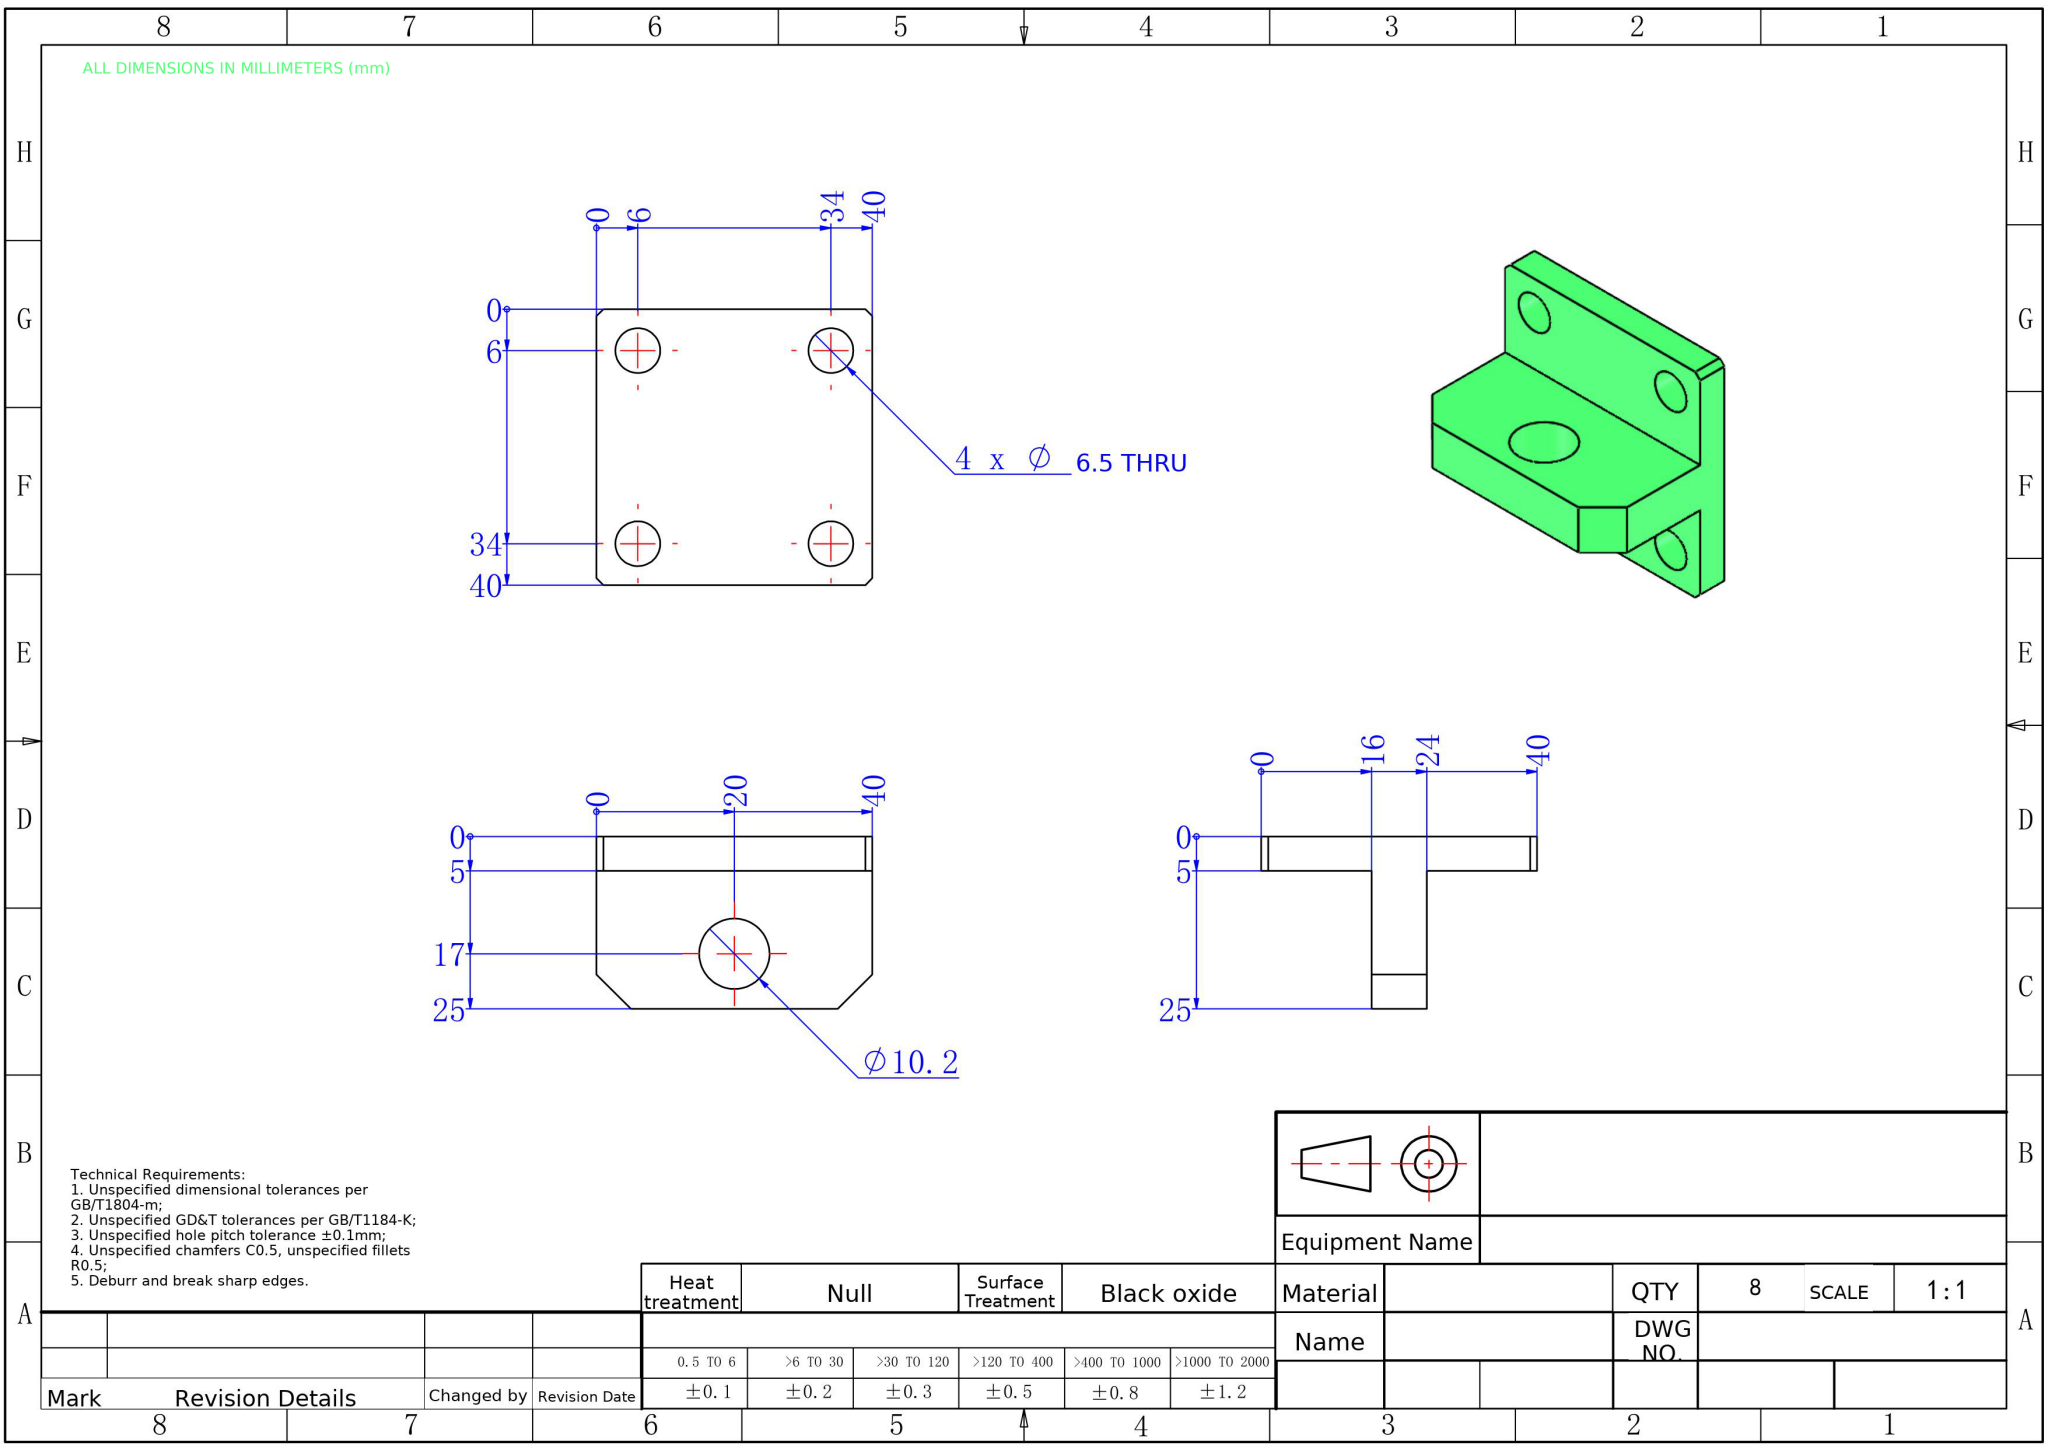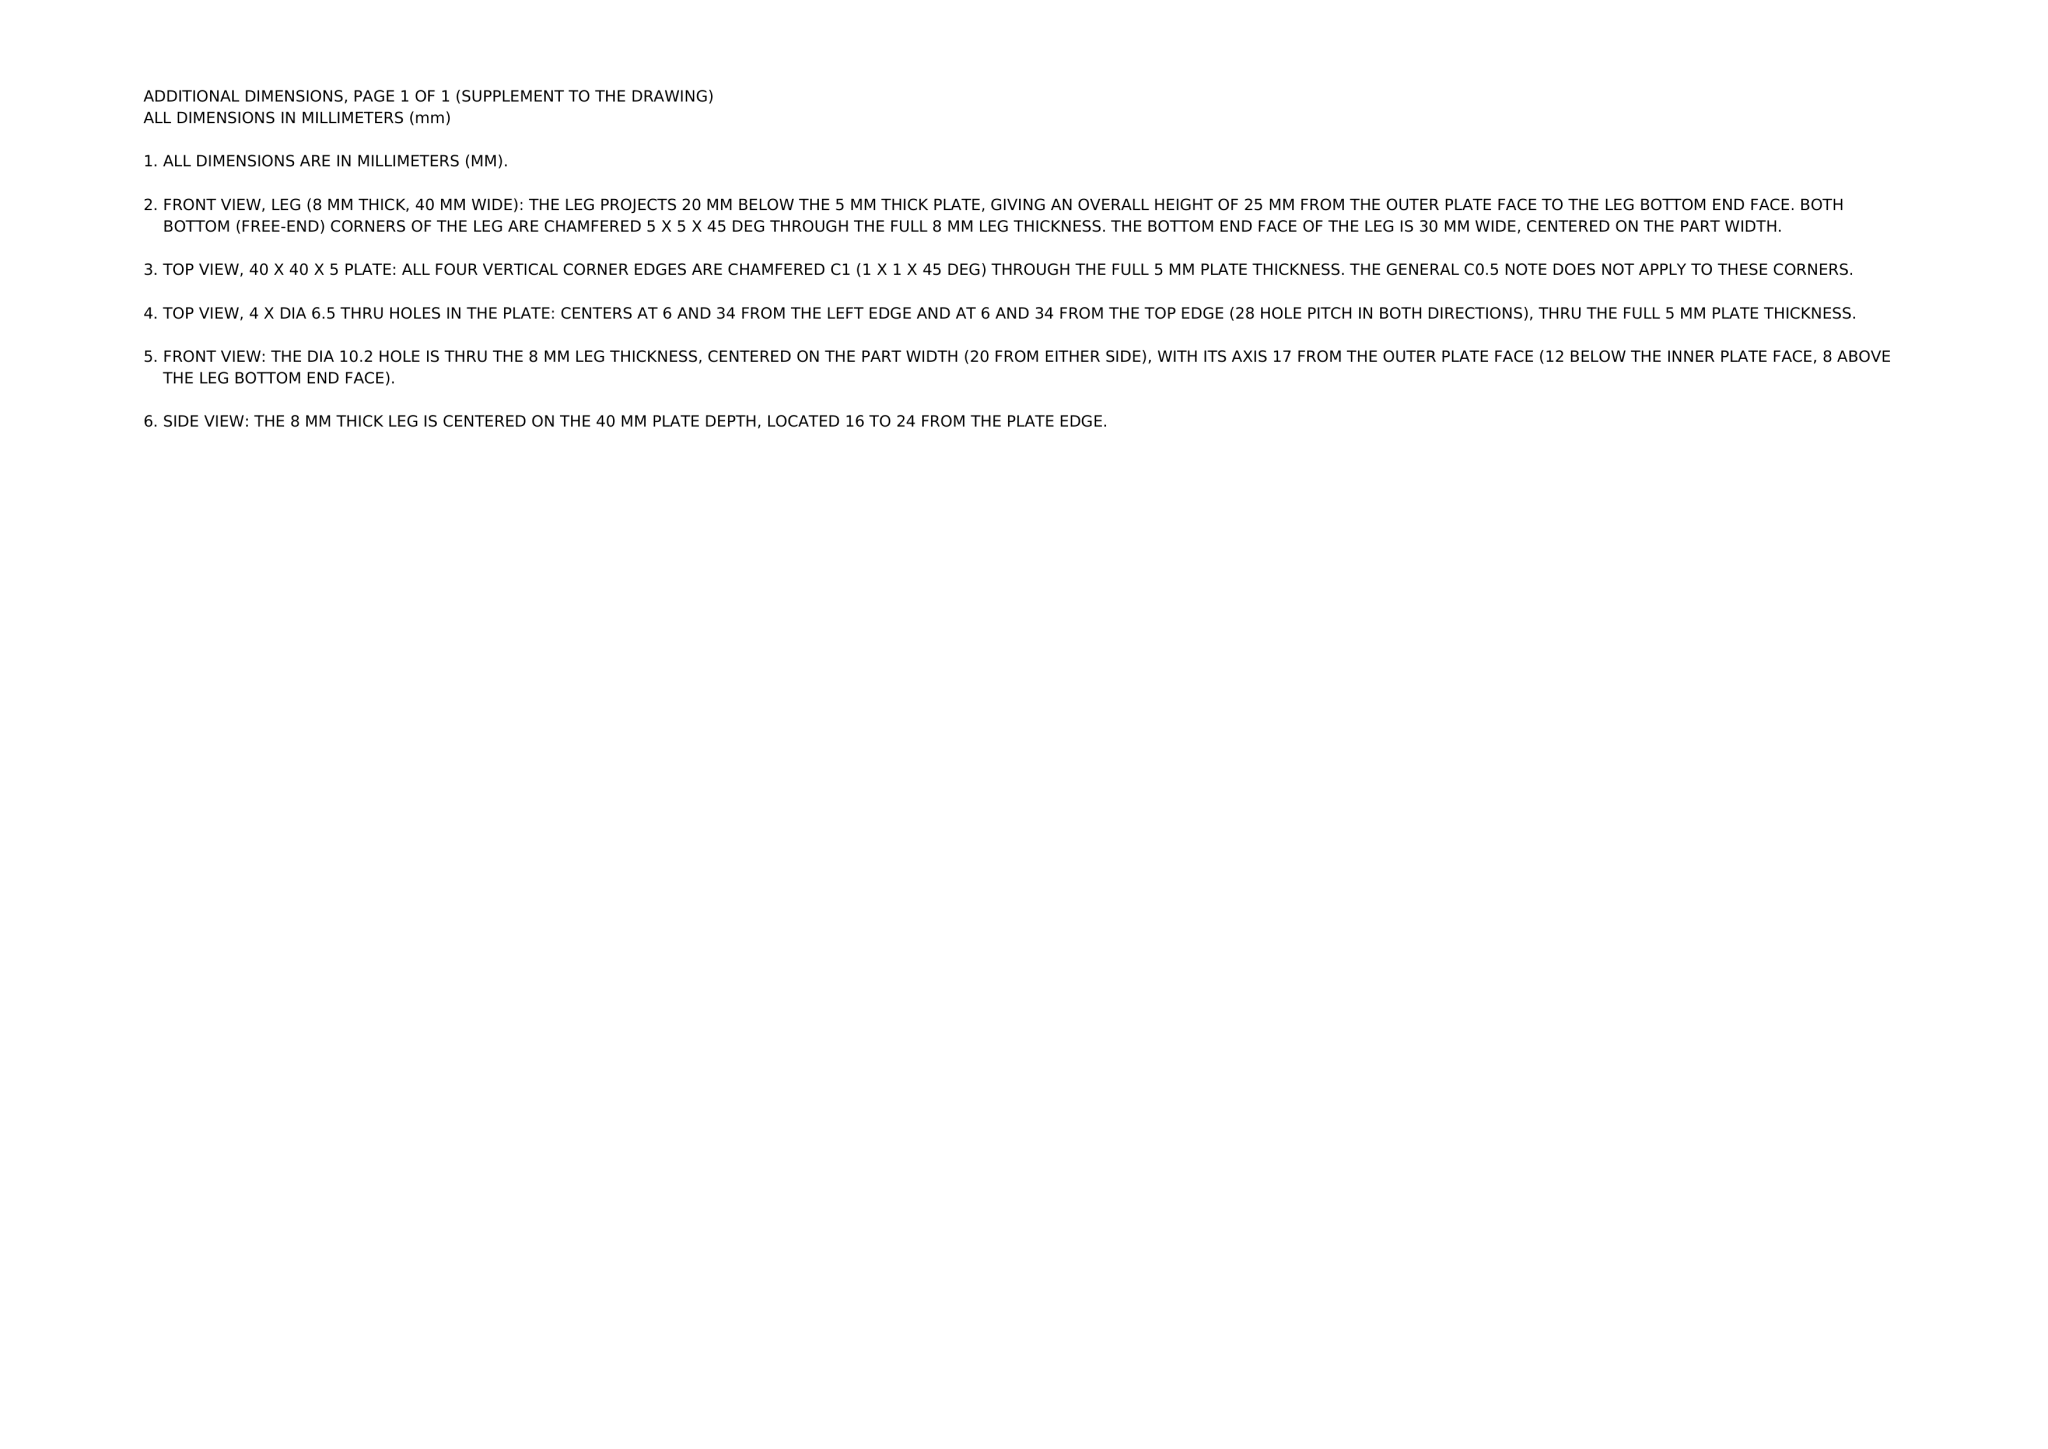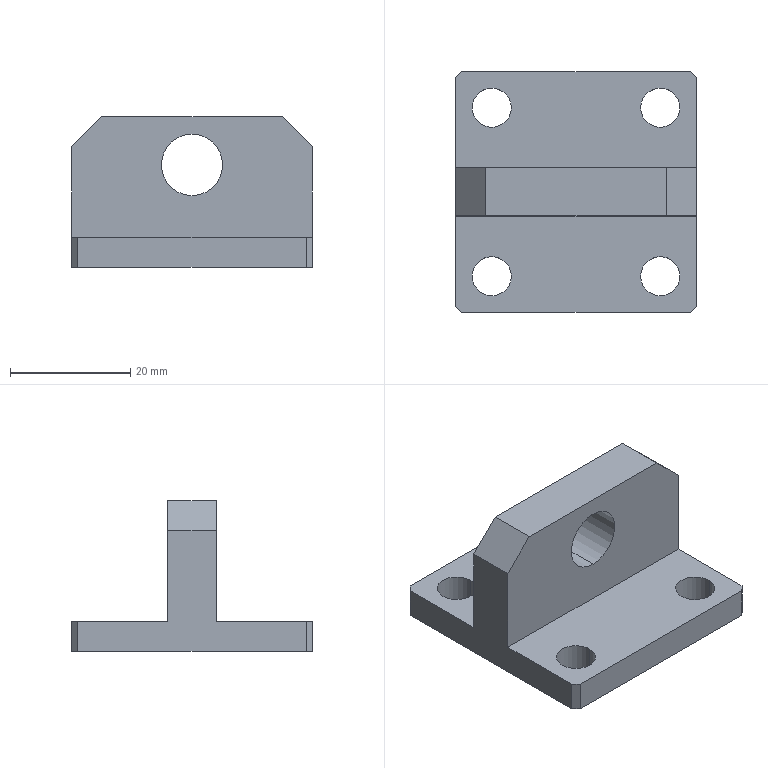Part | NX | mm | 1 solid | 26 faces | box 40 x 40 x 25 mm | volume 12873 mm3 | plane 16 | cylinder 10 | commonest cylinder face diameters 6.5 x8 10.2 x2
STEP:
#1=COLOUR_RGB('',0.7922,0.8196,0.9333);
#2=FILL_AREA_STYLE_COLOUR('',#1);
#3=FILL_AREA_STYLE('',(#2));
#4=SURFACE_STYLE_FILL_AREA(#3);
#5=SURFACE_SIDE_STYLE('',(#4));
#6=SURFACE_STYLE_USAGE(.BOTH.,#5);
#7=PRESENTATION_STYLE_ASSIGNMENT((#6));
#8=CARTESIAN_POINT('',(0.,-4.,11.9));
#9=VERTEX_POINT('',#8);
#10=CARTESIAN_POINT('',(0.,-4.,22.1));
#11=VERTEX_POINT('',#10);
#12=CARTESIAN_POINT('',(0.,-4.,17.));
#13=DIRECTION('',(0.,1.,0.));
#14=DIRECTION('',(0.,0.,1.));
#15=AXIS2_PLACEMENT_3D('',#12,#13,#14);
#16=CIRCLE('',#15,5.1);
#17=EDGE_CURVE('',#9,#11,#16,.T.);
#18=ORIENTED_EDGE('',*,*,#17,.F.);
#19=CARTESIAN_POINT('',(0.,4.,11.9));
#20=VERTEX_POINT('',#19);
#21=CARTESIAN_POINT('',(0.,-20.,11.9));
#22=DIRECTION('',(0.,1.,0.));
#23=VECTOR('',#22,1000.);
#24=LINE('',#21,#23);
#25=EDGE_CURVE('',#9,#20,#24,.T.);
#26=ORIENTED_EDGE('',*,*,#25,.T.);
#27=CARTESIAN_POINT('',(0.,4.,22.1));
#28=VERTEX_POINT('',#27);
#29=CARTESIAN_POINT('',(0.,4.,17.));
#30=DIRECTION('',(0.,1.,0.));
#31=DIRECTION('',(0.,0.,1.));
#32=AXIS2_PLACEMENT_3D('',#29,#30,#31);
#33=CIRCLE('',#32,5.1);
#34=EDGE_CURVE('',#20,#28,#33,.T.);
#35=ORIENTED_EDGE('',*,*,#34,.T.);
#36=CARTESIAN_POINT('',(0.,-20.,22.1));
#37=DIRECTION('',(0.,1.,0.));
#38=VECTOR('',#37,1000.);
#39=LINE('',#36,#38);
#40=EDGE_CURVE('',#11,#28,#39,.T.);
#41=ORIENTED_EDGE('',*,*,#40,.F.);
#42=EDGE_LOOP('',(#18,#26,#35,#41));
#43=FACE_OUTER_BOUND('',#42,.T.);
#44=CARTESIAN_POINT('',(0.,-20.,17.));
#45=DIRECTION('',(0.,1.,0.));
#46=DIRECTION('',(0.,0.,1.));
#47=AXIS2_PLACEMENT_3D('',#44,#45,#46);
#48=CYLINDRICAL_SURFACE('',#47,5.1);
#49=ADVANCED_FACE('',(#43),#48,.F.);
#50=CARTESIAN_POINT('',(10.75,-14.,0.));
#51=VERTEX_POINT('',#50);
#52=CARTESIAN_POINT('',(17.25,-14.,0.));
#53=VERTEX_POINT('',#52);
#54=CARTESIAN_POINT('',(14.,-14.,0.));
#55=DIRECTION('',(0.,0.,1.));
#56=DIRECTION('',(1.,0.,0.));
#57=AXIS2_PLACEMENT_3D('',#54,#55,#56);
#58=CIRCLE('',#57,3.25);
#59=EDGE_CURVE('',#51,#53,#58,.T.);
#60=ORIENTED_EDGE('',*,*,#59,.F.);
#61=CARTESIAN_POINT('',(10.75,-14.,5.));
#62=VERTEX_POINT('',#61);
#63=CARTESIAN_POINT('',(10.75,-14.,5.));
#64=DIRECTION('',(0.,0.,1.));
#65=VECTOR('',#64,1000.);
#66=LINE('',#63,#65);
#67=EDGE_CURVE('',#51,#62,#66,.T.);
#68=ORIENTED_EDGE('',*,*,#67,.T.);
#69=CARTESIAN_POINT('',(17.25,-14.,5.));
#70=VERTEX_POINT('',#69);
#71=CARTESIAN_POINT('',(14.,-14.,5.));
#72=DIRECTION('',(0.,0.,1.));
#73=DIRECTION('',(1.,0.,0.));
#74=AXIS2_PLACEMENT_3D('',#71,#72,#73);
#75=CIRCLE('',#74,3.25);
#76=EDGE_CURVE('',#62,#70,#75,.T.);
#77=ORIENTED_EDGE('',*,*,#76,.T.);
#78=CARTESIAN_POINT('',(17.25,-14.,5.));
#79=DIRECTION('',(0.,0.,1.));
#80=VECTOR('',#79,1000.);
#81=LINE('',#78,#80);
#82=EDGE_CURVE('',#53,#70,#81,.T.);
#83=ORIENTED_EDGE('',*,*,#82,.F.);
#84=EDGE_LOOP('',(#60,#68,#77,#83));
#85=FACE_OUTER_BOUND('',#84,.T.);
#86=CARTESIAN_POINT('',(14.,-14.,5.));
#87=DIRECTION('',(0.,0.,1.));
#88=DIRECTION('',(1.,0.,0.));
#89=AXIS2_PLACEMENT_3D('',#86,#87,#88);
#90=CYLINDRICAL_SURFACE('',#89,3.25);
#91=ADVANCED_FACE('',(#85),#90,.F.);
#92=CARTESIAN_POINT('',(-17.25,14.,0.));
#93=VERTEX_POINT('',#92);
#94=CARTESIAN_POINT('',(-10.75,14.,0.));
#95=VERTEX_POINT('',#94);
#96=CARTESIAN_POINT('',(-14.,14.,0.));
#97=DIRECTION('',(0.,0.,1.));
#98=DIRECTION('',(1.,0.,0.));
#99=AXIS2_PLACEMENT_3D('',#96,#97,#98);
#100=CIRCLE('',#99,3.25);
#101=EDGE_CURVE('',#93,#95,#100,.T.);
#102=ORIENTED_EDGE('',*,*,#101,.F.);
#103=CARTESIAN_POINT('',(-17.25,14.,5.));
#104=VERTEX_POINT('',#103);
#105=CARTESIAN_POINT('',(-17.25,14.,5.));
#106=DIRECTION('',(0.,0.,1.));
#107=VECTOR('',#106,1000.);
#108=LINE('',#105,#107);
#109=EDGE_CURVE('',#93,#104,#108,.T.);
#110=ORIENTED_EDGE('',*,*,#109,.T.);
#111=CARTESIAN_POINT('',(-10.75,14.,5.));
#112=VERTEX_POINT('',#111);
#113=CARTESIAN_POINT('',(-14.,14.,5.));
#114=DIRECTION('',(0.,0.,1.));
#115=DIRECTION('',(1.,0.,0.));
#116=AXIS2_PLACEMENT_3D('',#113,#114,#115);
#117=CIRCLE('',#116,3.25);
#118=EDGE_CURVE('',#104,#112,#117,.T.);
#119=ORIENTED_EDGE('',*,*,#118,.T.);
#120=CARTESIAN_POINT('',(-10.75,14.,5.));
#121=DIRECTION('',(0.,0.,1.));
#122=VECTOR('',#121,1000.);
#123=LINE('',#120,#122);
#124=EDGE_CURVE('',#95,#112,#123,.T.);
#125=ORIENTED_EDGE('',*,*,#124,.F.);
#126=EDGE_LOOP('',(#102,#110,#119,#125));
#127=FACE_OUTER_BOUND('',#126,.T.);
#128=CARTESIAN_POINT('',(-14.,14.,5.));
#129=DIRECTION('',(0.,0.,1.));
#130=DIRECTION('',(1.,0.,0.));
#131=AXIS2_PLACEMENT_3D('',#128,#129,#130);
#132=CYLINDRICAL_SURFACE('',#131,3.25);
#133=ADVANCED_FACE('',(#127),#132,.F.);
#134=CARTESIAN_POINT('',(-17.25,-14.,0.));
#135=VERTEX_POINT('',#134);
#136=CARTESIAN_POINT('',(-10.75,-14.,0.));
#137=VERTEX_POINT('',#136);
#138=CARTESIAN_POINT('',(-14.,-14.,0.));
#139=DIRECTION('',(0.,0.,1.));
#140=DIRECTION('',(1.,0.,0.));
#141=AXIS2_PLACEMENT_3D('',#138,#139,#140);
#142=CIRCLE('',#141,3.25);
#143=EDGE_CURVE('',#135,#137,#142,.T.);
#144=ORIENTED_EDGE('',*,*,#143,.F.);
#145=CARTESIAN_POINT('',(-17.25,-14.,5.));
#146=VERTEX_POINT('',#145);
#147=CARTESIAN_POINT('',(-17.25,-14.,5.));
#148=DIRECTION('',(0.,0.,1.));
#149=VECTOR('',#148,1000.);
#150=LINE('',#147,#149);
#151=EDGE_CURVE('',#135,#146,#150,.T.);
#152=ORIENTED_EDGE('',*,*,#151,.T.);
#153=CARTESIAN_POINT('',(-10.75,-14.,5.));
#154=VERTEX_POINT('',#153);
#155=CARTESIAN_POINT('',(-14.,-14.,5.));
#156=DIRECTION('',(0.,0.,1.));
#157=DIRECTION('',(1.,0.,0.));
#158=AXIS2_PLACEMENT_3D('',#155,#156,#157);
#159=CIRCLE('',#158,3.25);
#160=EDGE_CURVE('',#146,#154,#159,.T.);
#161=ORIENTED_EDGE('',*,*,#160,.T.);
#162=CARTESIAN_POINT('',(-10.75,-14.,5.));
#163=DIRECTION('',(0.,0.,1.));
#164=VECTOR('',#163,1000.);
#165=LINE('',#162,#164);
#166=EDGE_CURVE('',#137,#154,#165,.T.);
#167=ORIENTED_EDGE('',*,*,#166,.F.);
#168=EDGE_LOOP('',(#144,#152,#161,#167));
#169=FACE_OUTER_BOUND('',#168,.T.);
#170=CARTESIAN_POINT('',(-14.,-14.,5.));
#171=DIRECTION('',(0.,0.,1.));
#172=DIRECTION('',(1.,0.,0.));
#173=AXIS2_PLACEMENT_3D('',#170,#171,#172);
#174=CYLINDRICAL_SURFACE('',#173,3.25);
#175=ADVANCED_FACE('',(#169),#174,.F.);
#176=CARTESIAN_POINT('',(10.75,14.,0.));
#177=VERTEX_POINT('',#176);
#178=CARTESIAN_POINT('',(17.25,14.,0.));
#179=VERTEX_POINT('',#178);
#180=CARTESIAN_POINT('',(14.,14.,0.));
#181=DIRECTION('',(0.,0.,1.));
#182=DIRECTION('',(1.,0.,0.));
#183=AXIS2_PLACEMENT_3D('',#180,#181,#182);
#184=CIRCLE('',#183,3.25);
#185=EDGE_CURVE('',#177,#179,#184,.T.);
#186=ORIENTED_EDGE('',*,*,#185,.F.);
#187=CARTESIAN_POINT('',(10.75,14.,5.));
#188=VERTEX_POINT('',#187);
#189=CARTESIAN_POINT('',(10.75,14.,5.));
#190=DIRECTION('',(0.,0.,1.));
#191=VECTOR('',#190,1000.);
#192=LINE('',#189,#191);
#193=EDGE_CURVE('',#177,#188,#192,.T.);
#194=ORIENTED_EDGE('',*,*,#193,.T.);
#195=CARTESIAN_POINT('',(17.25,14.,5.));
#196=VERTEX_POINT('',#195);
#197=CARTESIAN_POINT('',(14.,14.,5.));
#198=DIRECTION('',(0.,0.,1.));
#199=DIRECTION('',(1.,0.,0.));
#200=AXIS2_PLACEMENT_3D('',#197,#198,#199);
#201=CIRCLE('',#200,3.25);
#202=EDGE_CURVE('',#188,#196,#201,.T.);
#203=ORIENTED_EDGE('',*,*,#202,.T.);
#204=CARTESIAN_POINT('',(17.25,14.,5.));
#205=DIRECTION('',(0.,0.,1.));
#206=VECTOR('',#205,1000.);
#207=LINE('',#204,#206);
#208=EDGE_CURVE('',#179,#196,#207,.T.);
#209=ORIENTED_EDGE('',*,*,#208,.F.);
#210=EDGE_LOOP('',(#186,#194,#203,#209));
#211=FACE_OUTER_BOUND('',#210,.T.);
#212=CARTESIAN_POINT('',(14.,14.,5.));
#213=DIRECTION('',(0.,0.,1.));
#214=DIRECTION('',(1.,0.,0.));
#215=AXIS2_PLACEMENT_3D('',#212,#213,#214);
#216=CYLINDRICAL_SURFACE('',#215,3.25);
#217=ADVANCED_FACE('',(#211),#216,.F.);
#218=CARTESIAN_POINT('',(-20.,-4.,5.));
#219=VERTEX_POINT('',#218);
#220=CARTESIAN_POINT('',(20.,-4.,5.));
#221=VERTEX_POINT('',#220);
#222=CARTESIAN_POINT('',(-20.,-4.,5.));
#223=DIRECTION('',(1.,0.,0.));
#224=VECTOR('',#223,1000.);
#225=LINE('',#222,#224);
#226=EDGE_CURVE('',#219,#221,#225,.T.);
#227=ORIENTED_EDGE('',*,*,#226,.F.);
#228=CARTESIAN_POINT('',(-20.,-19.,5.));
#229=VERTEX_POINT('',#228);
#230=CARTESIAN_POINT('',(-20.,20.,5.));
#231=DIRECTION('',(0.,-1.,0.));
#232=VECTOR('',#231,1000.);
#233=LINE('',#230,#232);
#234=EDGE_CURVE('',#219,#229,#233,.T.);
#235=ORIENTED_EDGE('',*,*,#234,.T.);
#236=CARTESIAN_POINT('',(-19.,-20.,5.));
#237=VERTEX_POINT('',#236);
#238=CARTESIAN_POINT('',(-19.5,-19.5,5.));
#239=DIRECTION('',(0.7071,-0.7071,0.));
#240=VECTOR('',#239,1000.);
#241=LINE('',#238,#240);
#242=EDGE_CURVE('',#229,#237,#241,.T.);
#243=ORIENTED_EDGE('',*,*,#242,.T.);
#244=CARTESIAN_POINT('',(19.,-20.,5.));
#245=VERTEX_POINT('',#244);
#246=CARTESIAN_POINT('',(-20.,-20.,5.));
#247=DIRECTION('',(1.,0.,0.));
#248=VECTOR('',#247,1000.);
#249=LINE('',#246,#248);
#250=EDGE_CURVE('',#237,#245,#249,.T.);
#251=ORIENTED_EDGE('',*,*,#250,.T.);
#252=CARTESIAN_POINT('',(20.,-19.,5.));
#253=VERTEX_POINT('',#252);
#254=CARTESIAN_POINT('',(19.5,-19.5,5.));
#255=DIRECTION('',(0.7071,0.7071,0.));
#256=VECTOR('',#255,1000.);
#257=LINE('',#254,#256);
#258=EDGE_CURVE('',#245,#253,#257,.T.);
#259=ORIENTED_EDGE('',*,*,#258,.T.);
#260=CARTESIAN_POINT('',(20.,20.,5.));
#261=DIRECTION('',(-0.,1.,0.));
#262=VECTOR('',#261,1000.);
#263=LINE('',#260,#262);
#264=EDGE_CURVE('',#253,#221,#263,.T.);
#265=ORIENTED_EDGE('',*,*,#264,.T.);
#266=EDGE_LOOP('',(#227,#235,#243,#251,#259,#265));
#267=FACE_OUTER_BOUND('',#266,.T.);
#268=CARTESIAN_POINT('',(-14.,-14.,5.));
#269=DIRECTION('',(0.,0.,1.));
#270=DIRECTION('',(1.,0.,0.));
#271=AXIS2_PLACEMENT_3D('',#268,#269,#270);
#272=CIRCLE('',#271,3.25);
#273=EDGE_CURVE('',#154,#146,#272,.T.);
#274=ORIENTED_EDGE('',*,*,#273,.F.);
#275=ORIENTED_EDGE('',*,*,#160,.F.);
#276=EDGE_LOOP('',(#274,#275));
#277=FACE_BOUND('',#276,.T.);
#278=CARTESIAN_POINT('',(14.,-14.,5.));
#279=DIRECTION('',(0.,0.,1.));
#280=DIRECTION('',(1.,0.,0.));
#281=AXIS2_PLACEMENT_3D('',#278,#279,#280);
#282=CIRCLE('',#281,3.25);
#283=EDGE_CURVE('',#70,#62,#282,.T.);
#284=ORIENTED_EDGE('',*,*,#283,.F.);
#285=ORIENTED_EDGE('',*,*,#76,.F.);
#286=EDGE_LOOP('',(#284,#285));
#287=FACE_BOUND('',#286,.T.);
#288=CARTESIAN_POINT('',(0.,0.,5.));
#289=DIRECTION('',(0.,0.,1.));
#290=DIRECTION('',(1.,0.,0.));
#291=AXIS2_PLACEMENT_3D('',#288,#289,#290);
#292=PLANE('',#291);
#293=ADVANCED_FACE('',(#267,#277,#287),#292,.T.);
#294=CARTESIAN_POINT('',(20.,4.,20.));
#295=VERTEX_POINT('',#294);
#296=CARTESIAN_POINT('',(20.,4.,5.));
#297=VERTEX_POINT('',#296);
#298=CARTESIAN_POINT('',(20.,4.,25.));
#299=DIRECTION('',(0.,0.,-1.));
#300=VECTOR('',#299,1000.);
#301=LINE('',#298,#300);
#302=EDGE_CURVE('',#295,#297,#301,.T.);
#303=ORIENTED_EDGE('',*,*,#302,.F.);
#304=CARTESIAN_POINT('',(20.,-4.,20.));
#305=VERTEX_POINT('',#304);
#306=CARTESIAN_POINT('',(20.,-4.,20.));
#307=DIRECTION('',(0.,-1.,0.));
#308=VECTOR('',#307,1000.);
#309=LINE('',#306,#308);
#310=EDGE_CURVE('',#295,#305,#309,.T.);
#311=ORIENTED_EDGE('',*,*,#310,.T.);
#312=CARTESIAN_POINT('',(20.,-4.,25.));
#313=DIRECTION('',(0.,0.,-1.));
#314=VECTOR('',#313,1000.);
#315=LINE('',#312,#314);
#316=EDGE_CURVE('',#305,#221,#315,.T.);
#317=ORIENTED_EDGE('',*,*,#316,.T.);
#318=ORIENTED_EDGE('',*,*,#264,.F.);
#319=CARTESIAN_POINT('',(20.,-19.,0.));
#320=VERTEX_POINT('',#319);
#321=CARTESIAN_POINT('',(20.,-19.,5.));
#322=DIRECTION('',(0.,0.,-1.));
#323=VECTOR('',#322,1000.);
#324=LINE('',#321,#323);
#325=EDGE_CURVE('',#253,#320,#324,.T.);
#326=ORIENTED_EDGE('',*,*,#325,.T.);
#327=CARTESIAN_POINT('',(20.,19.,0.));
#328=VERTEX_POINT('',#327);
#329=CARTESIAN_POINT('',(20.,20.,0.));
#330=DIRECTION('',(-0.,1.,0.));
#331=VECTOR('',#330,1000.);
#332=LINE('',#329,#331);
#333=EDGE_CURVE('',#320,#328,#332,.T.);
#334=ORIENTED_EDGE('',*,*,#333,.T.);
#335=CARTESIAN_POINT('',(20.,19.,5.));
#336=VERTEX_POINT('',#335);
#337=CARTESIAN_POINT('',(20.,19.,5.));
#338=DIRECTION('',(0.,0.,1.));
#339=VECTOR('',#338,1000.);
#340=LINE('',#337,#339);
#341=EDGE_CURVE('',#328,#336,#340,.T.);
#342=ORIENTED_EDGE('',*,*,#341,.T.);
#343=CARTESIAN_POINT('',(20.,20.,5.));
#344=DIRECTION('',(-0.,1.,0.));
#345=VECTOR('',#344,1000.);
#346=LINE('',#343,#345);
#347=EDGE_CURVE('',#297,#336,#346,.T.);
#348=ORIENTED_EDGE('',*,*,#347,.F.);
#349=EDGE_LOOP('',(#303,#311,#317,#318,#326,#334,#342,#348));
#350=FACE_OUTER_BOUND('',#349,.T.);
#351=CARTESIAN_POINT('',(20.,20.,5.));
#352=DIRECTION('',(-1.,-0.,0.));
#353=DIRECTION('',(0.,-1.,0.));
#354=AXIS2_PLACEMENT_3D('',#351,#352,#353);
#355=PLANE('',#354);
#356=ADVANCED_FACE('',(#350),#355,.F.);
#357=CARTESIAN_POINT('',(19.,20.,0.));
#358=VERTEX_POINT('',#357);
#359=CARTESIAN_POINT('',(-19.,20.,0.));
#360=VERTEX_POINT('',#359);
#361=CARTESIAN_POINT('',(-20.,20.,0.));
#362=DIRECTION('',(-1.,0.,0.));
#363=VECTOR('',#362,1000.);
#364=LINE('',#361,#363);
#365=EDGE_CURVE('',#358,#360,#364,.T.);
#366=ORIENTED_EDGE('',*,*,#365,.T.);
#367=CARTESIAN_POINT('',(-19.,20.,5.));
#368=VERTEX_POINT('',#367);
#369=CARTESIAN_POINT('',(-19.,20.,5.));
#370=DIRECTION('',(0.,0.,1.));
#371=VECTOR('',#370,1000.);
#372=LINE('',#369,#371);
#373=EDGE_CURVE('',#360,#368,#372,.T.);
#374=ORIENTED_EDGE('',*,*,#373,.T.);
#375=CARTESIAN_POINT('',(19.,20.,5.));
#376=VERTEX_POINT('',#375);
#377=CARTESIAN_POINT('',(-20.,20.,5.));
#378=DIRECTION('',(-1.,0.,0.));
#379=VECTOR('',#378,1000.);
#380=LINE('',#377,#379);
#381=EDGE_CURVE('',#376,#368,#380,.T.);
#382=ORIENTED_EDGE('',*,*,#381,.F.);
#383=CARTESIAN_POINT('',(19.,20.,5.));
#384=DIRECTION('',(0.,0.,-1.));
#385=VECTOR('',#384,1000.);
#386=LINE('',#383,#385);
#387=EDGE_CURVE('',#376,#358,#386,.T.);
#388=ORIENTED_EDGE('',*,*,#387,.T.);
#389=EDGE_LOOP('',(#366,#374,#382,#388));
#390=FACE_OUTER_BOUND('',#389,.T.);
#391=CARTESIAN_POINT('',(-20.,20.,5.));
#392=DIRECTION('',(0.,-1.,0.));
#393=DIRECTION('',(0.,0.,-1.));
#394=AXIS2_PLACEMENT_3D('',#391,#392,#393);
#395=PLANE('',#394);
#396=ADVANCED_FACE('',(#390),#395,.F.);
#397=CARTESIAN_POINT('',(-20.,-4.,20.));
#398=VERTEX_POINT('',#397);
#399=CARTESIAN_POINT('',(-20.,-4.,25.));
#400=DIRECTION('',(0.,0.,-1.));
#401=VECTOR('',#400,1000.);
#402=LINE('',#399,#401);
#403=EDGE_CURVE('',#398,#219,#402,.T.);
#404=ORIENTED_EDGE('',*,*,#403,.F.);
#405=CARTESIAN_POINT('',(-20.,4.,20.));
#406=VERTEX_POINT('',#405);
#407=CARTESIAN_POINT('',(-20.,4.,20.));
#408=DIRECTION('',(-0.,1.,0.));
#409=VECTOR('',#408,1000.);
#410=LINE('',#407,#409);
#411=EDGE_CURVE('',#398,#406,#410,.T.);
#412=ORIENTED_EDGE('',*,*,#411,.T.);
#413=CARTESIAN_POINT('',(-20.,4.,5.));
#414=VERTEX_POINT('',#413);
#415=CARTESIAN_POINT('',(-20.,4.,25.));
#416=DIRECTION('',(0.,0.,-1.));
#417=VECTOR('',#416,1000.);
#418=LINE('',#415,#417);
#419=EDGE_CURVE('',#406,#414,#418,.T.);
#420=ORIENTED_EDGE('',*,*,#419,.T.);
#421=CARTESIAN_POINT('',(-20.,19.,5.));
#422=VERTEX_POINT('',#421);
#423=CARTESIAN_POINT('',(-20.,20.,5.));
#424=DIRECTION('',(0.,-1.,0.));
#425=VECTOR('',#424,1000.);
#426=LINE('',#423,#425);
#427=EDGE_CURVE('',#422,#414,#426,.T.);
#428=ORIENTED_EDGE('',*,*,#427,.F.);
#429=CARTESIAN_POINT('',(-20.,19.,0.));
#430=VERTEX_POINT('',#429);
#431=CARTESIAN_POINT('',(-20.,19.,5.));
#432=DIRECTION('',(0.,0.,-1.));
#433=VECTOR('',#432,1000.);
#434=LINE('',#431,#433);
#435=EDGE_CURVE('',#422,#430,#434,.T.);
#436=ORIENTED_EDGE('',*,*,#435,.T.);
#437=CARTESIAN_POINT('',(-20.,-19.,0.));
#438=VERTEX_POINT('',#437);
#439=CARTESIAN_POINT('',(-20.,20.,0.));
#440=DIRECTION('',(0.,-1.,0.));
#441=VECTOR('',#440,1000.);
#442=LINE('',#439,#441);
#443=EDGE_CURVE('',#430,#438,#442,.T.);
#444=ORIENTED_EDGE('',*,*,#443,.T.);
#445=CARTESIAN_POINT('',(-20.,-19.,5.));
#446=DIRECTION('',(0.,0.,1.));
#447=VECTOR('',#446,1000.);
#448=LINE('',#445,#447);
#449=EDGE_CURVE('',#438,#229,#448,.T.);
#450=ORIENTED_EDGE('',*,*,#449,.T.);
#451=ORIENTED_EDGE('',*,*,#234,.F.);
#452=EDGE_LOOP('',(#404,#412,#420,#428,#436,#444,#450,#451));
#453=FACE_OUTER_BOUND('',#452,.T.);
#454=CARTESIAN_POINT('',(-20.,20.,5.));
#455=DIRECTION('',(1.,0.,0.));
#456=DIRECTION('',(-0.,1.,0.));
#457=AXIS2_PLACEMENT_3D('',#454,#455,#456);
#458=PLANE('',#457);
#459=ADVANCED_FACE('',(#453),#458,.F.);
#460=ORIENTED_EDGE('',*,*,#250,.F.);
#461=CARTESIAN_POINT('',(-19.,-20.,0.));
#462=VERTEX_POINT('',#461);
#463=CARTESIAN_POINT('',(-19.,-20.,5.));
#464=DIRECTION('',(0.,0.,-1.));
#465=VECTOR('',#464,1000.);
#466=LINE('',#463,#465);
#467=EDGE_CURVE('',#237,#462,#466,.T.);
#468=ORIENTED_EDGE('',*,*,#467,.T.);
#469=CARTESIAN_POINT('',(19.,-20.,0.));
#470=VERTEX_POINT('',#469);
#471=CARTESIAN_POINT('',(-20.,-20.,0.));
#472=DIRECTION('',(1.,0.,0.));
#473=VECTOR('',#472,1000.);
#474=LINE('',#471,#473);
#475=EDGE_CURVE('',#462,#470,#474,.T.);
#476=ORIENTED_EDGE('',*,*,#475,.T.);
#477=CARTESIAN_POINT('',(19.,-20.,5.));
#478=DIRECTION('',(0.,0.,1.));
#479=VECTOR('',#478,1000.);
#480=LINE('',#477,#479);
#481=EDGE_CURVE('',#470,#245,#480,.T.);
#482=ORIENTED_EDGE('',*,*,#481,.T.);
#483=EDGE_LOOP('',(#460,#468,#476,#482));
#484=FACE_OUTER_BOUND('',#483,.T.);
#485=CARTESIAN_POINT('',(-20.,-20.,5.));
#486=DIRECTION('',(0.,1.,0.));
#487=DIRECTION('',(0.,0.,1.));
#488=AXIS2_PLACEMENT_3D('',#485,#486,#487);
#489=PLANE('',#488);
#490=ADVANCED_FACE('',(#484),#489,.F.);
#491=CARTESIAN_POINT('',(-20.,4.,5.));
#492=DIRECTION('',(-1.,0.,0.));
#493=VECTOR('',#492,1000.);
#494=LINE('',#491,#493);
#495=EDGE_CURVE('',#297,#414,#494,.T.);
#496=ORIENTED_EDGE('',*,*,#495,.F.);
#497=ORIENTED_EDGE('',*,*,#347,.T.);
#498=CARTESIAN_POINT('',(19.5,19.5,5.));
#499=DIRECTION('',(-0.7071,0.7071,0.));
#500=VECTOR('',#499,1000.);
#501=LINE('',#498,#500);
#502=EDGE_CURVE('',#336,#376,#501,.T.);
#503=ORIENTED_EDGE('',*,*,#502,.T.);
#504=ORIENTED_EDGE('',*,*,#381,.T.);
#505=CARTESIAN_POINT('',(-19.5,19.5,5.));
#506=DIRECTION('',(-0.7071,-0.7071,0.));
#507=VECTOR('',#506,1000.);
#508=LINE('',#505,#507);
#509=EDGE_CURVE('',#368,#422,#508,.T.);
#510=ORIENTED_EDGE('',*,*,#509,.T.);
#511=ORIENTED_EDGE('',*,*,#427,.T.);
#512=EDGE_LOOP('',(#496,#497,#503,#504,#510,#511));
#513=FACE_OUTER_BOUND('',#512,.T.);
#514=CARTESIAN_POINT('',(-14.,14.,5.));
#515=DIRECTION('',(0.,0.,1.));
#516=DIRECTION('',(1.,0.,0.));
#517=AXIS2_PLACEMENT_3D('',#514,#515,#516);
#518=CIRCLE('',#517,3.25);
#519=EDGE_CURVE('',#112,#104,#518,.T.);
#520=ORIENTED_EDGE('',*,*,#519,.F.);
#521=ORIENTED_EDGE('',*,*,#118,.F.);
#522=EDGE_LOOP('',(#520,#521));
#523=FACE_BOUND('',#522,.T.);
#524=CARTESIAN_POINT('',(14.,14.,5.));
#525=DIRECTION('',(0.,0.,1.));
#526=DIRECTION('',(1.,0.,0.));
#527=AXIS2_PLACEMENT_3D('',#524,#525,#526);
#528=CIRCLE('',#527,3.25);
#529=EDGE_CURVE('',#196,#188,#528,.T.);
#530=ORIENTED_EDGE('',*,*,#529,.F.);
#531=ORIENTED_EDGE('',*,*,#202,.F.);
#532=EDGE_LOOP('',(#530,#531));
#533=FACE_BOUND('',#532,.T.);
#534=CARTESIAN_POINT('',(0.,0.,5.));
#535=DIRECTION('',(0.,0.,1.));
#536=DIRECTION('',(1.,0.,0.));
#537=AXIS2_PLACEMENT_3D('',#534,#535,#536);
#538=PLANE('',#537);
#539=ADVANCED_FACE('',(#513,#523,#533),#538,.T.);
#540=CARTESIAN_POINT('',(14.,-14.,0.));
#541=DIRECTION('',(0.,0.,1.));
#542=DIRECTION('',(1.,0.,0.));
#543=AXIS2_PLACEMENT_3D('',#540,#541,#542);
#544=CIRCLE('',#543,3.25);
#545=EDGE_CURVE('',#53,#51,#544,.T.);
#546=ORIENTED_EDGE('',*,*,#545,.T.);
#547=ORIENTED_EDGE('',*,*,#59,.T.);
#548=EDGE_LOOP('',(#546,#547));
#549=FACE_BOUND('',#548,.T.);
#550=CARTESIAN_POINT('',(-14.,14.,0.));
#551=DIRECTION('',(0.,0.,1.));
#552=DIRECTION('',(1.,0.,0.));
#553=AXIS2_PLACEMENT_3D('',#550,#551,#552);
#554=CIRCLE('',#553,3.25);
#555=EDGE_CURVE('',#95,#93,#554,.T.);
#556=ORIENTED_EDGE('',*,*,#555,.T.);
#557=ORIENTED_EDGE('',*,*,#101,.T.);
#558=EDGE_LOOP('',(#556,#557));
#559=FACE_BOUND('',#558,.T.);
#560=CARTESIAN_POINT('',(-14.,-14.,0.));
#561=DIRECTION('',(0.,0.,1.));
#562=DIRECTION('',(1.,0.,0.));
#563=AXIS2_PLACEMENT_3D('',#560,#561,#562);
#564=CIRCLE('',#563,3.25);
#565=EDGE_CURVE('',#137,#135,#564,.T.);
#566=ORIENTED_EDGE('',*,*,#565,.T.);
#567=ORIENTED_EDGE('',*,*,#143,.T.);
#568=EDGE_LOOP('',(#566,#567));
#569=FACE_BOUND('',#568,.T.);
#570=CARTESIAN_POINT('',(14.,14.,0.));
#571=DIRECTION('',(0.,0.,1.));
#572=DIRECTION('',(1.,0.,0.));
#573=AXIS2_PLACEMENT_3D('',#570,#571,#572);
#574=CIRCLE('',#573,3.25);
#575=EDGE_CURVE('',#179,#177,#574,.T.);
#576=ORIENTED_EDGE('',*,*,#575,.T.);
#577=ORIENTED_EDGE('',*,*,#185,.T.);
#578=EDGE_LOOP('',(#576,#577));
#579=FACE_BOUND('',#578,.T.);
#580=ORIENTED_EDGE('',*,*,#475,.F.);
#581=CARTESIAN_POINT('',(-19.,-20.,0.));
#582=DIRECTION('',(-0.7071,0.7071,0.));
#583=VECTOR('',#582,1000.);
#584=LINE('',#581,#583);
#585=EDGE_CURVE('',#462,#438,#584,.T.);
#586=ORIENTED_EDGE('',*,*,#585,.T.);
#587=ORIENTED_EDGE('',*,*,#443,.F.);
#588=CARTESIAN_POINT('',(-20.,19.,0.));
#589=DIRECTION('',(0.7071,0.7071,0.));
#590=VECTOR('',#589,1000.);
#591=LINE('',#588,#590);
#592=EDGE_CURVE('',#430,#360,#591,.T.);
#593=ORIENTED_EDGE('',*,*,#592,.T.);
#594=ORIENTED_EDGE('',*,*,#365,.F.);
#595=CARTESIAN_POINT('',(19.,20.,0.));
#596=DIRECTION('',(0.7071,-0.7071,0.));
#597=VECTOR('',#596,1000.);
#598=LINE('',#595,#597);
#599=EDGE_CURVE('',#358,#328,#598,.T.);
#600=ORIENTED_EDGE('',*,*,#599,.T.);
#601=ORIENTED_EDGE('',*,*,#333,.F.);
#602=CARTESIAN_POINT('',(20.,-19.,0.));
#603=DIRECTION('',(-0.7071,-0.7071,0.));
#604=VECTOR('',#603,1000.);
#605=LINE('',#602,#604);
#606=EDGE_CURVE('',#320,#470,#605,.T.);
#607=ORIENTED_EDGE('',*,*,#606,.T.);
#608=EDGE_LOOP('',(#580,#586,#587,#593,#594,#600,#601,#607));
#609=FACE_OUTER_BOUND('',#608,.T.);
#610=CARTESIAN_POINT('',(0.,0.,0.));
#611=DIRECTION('',(0.,0.,1.));
#612=DIRECTION('',(1.,0.,0.));
#613=AXIS2_PLACEMENT_3D('',#610,#611,#612);
#614=PLANE('',#613);
#615=ADVANCED_FACE('',(#549,#559,#569,#579,#609),#614,.F.);
#616=ORIENTED_EDGE('',*,*,#193,.F.);
#617=ORIENTED_EDGE('',*,*,#575,.F.);
#618=ORIENTED_EDGE('',*,*,#208,.T.);
#619=ORIENTED_EDGE('',*,*,#529,.T.);
#620=EDGE_LOOP('',(#616,#617,#618,#619));
#621=FACE_OUTER_BOUND('',#620,.T.);
#622=CARTESIAN_POINT('',(14.,14.,5.));
#623=DIRECTION('',(0.,0.,1.));
#624=DIRECTION('',(1.,0.,0.));
#625=AXIS2_PLACEMENT_3D('',#622,#623,#624);
#626=CYLINDRICAL_SURFACE('',#625,3.25);
#627=ADVANCED_FACE('',(#621),#626,.F.);
#628=ORIENTED_EDGE('',*,*,#151,.F.);
#629=ORIENTED_EDGE('',*,*,#565,.F.);
#630=ORIENTED_EDGE('',*,*,#166,.T.);
#631=ORIENTED_EDGE('',*,*,#273,.T.);
#632=EDGE_LOOP('',(#628,#629,#630,#631));
#633=FACE_OUTER_BOUND('',#632,.T.);
#634=CARTESIAN_POINT('',(-14.,-14.,5.));
#635=DIRECTION('',(0.,0.,1.));
#636=DIRECTION('',(1.,0.,0.));
#637=AXIS2_PLACEMENT_3D('',#634,#635,#636);
#638=CYLINDRICAL_SURFACE('',#637,3.25);
#639=ADVANCED_FACE('',(#633),#638,.F.);
#640=ORIENTED_EDGE('',*,*,#109,.F.);
#641=ORIENTED_EDGE('',*,*,#555,.F.);
#642=ORIENTED_EDGE('',*,*,#124,.T.);
#643=ORIENTED_EDGE('',*,*,#519,.T.);
#644=EDGE_LOOP('',(#640,#641,#642,#643));
#645=FACE_OUTER_BOUND('',#644,.T.);
#646=CARTESIAN_POINT('',(-14.,14.,5.));
#647=DIRECTION('',(0.,0.,1.));
#648=DIRECTION('',(1.,0.,0.));
#649=AXIS2_PLACEMENT_3D('',#646,#647,#648);
#650=CYLINDRICAL_SURFACE('',#649,3.25);
#651=ADVANCED_FACE('',(#645),#650,.F.);
#652=ORIENTED_EDGE('',*,*,#67,.F.);
#653=ORIENTED_EDGE('',*,*,#545,.F.);
#654=ORIENTED_EDGE('',*,*,#82,.T.);
#655=ORIENTED_EDGE('',*,*,#283,.T.);
#656=EDGE_LOOP('',(#652,#653,#654,#655));
#657=FACE_OUTER_BOUND('',#656,.T.);
#658=CARTESIAN_POINT('',(14.,-14.,5.));
#659=DIRECTION('',(0.,0.,1.));
#660=DIRECTION('',(1.,0.,0.));
#661=AXIS2_PLACEMENT_3D('',#658,#659,#660);
#662=CYLINDRICAL_SURFACE('',#661,3.25);
#663=ADVANCED_FACE('',(#657),#662,.F.);
#664=ORIENTED_EDGE('',*,*,#242,.F.);
#665=ORIENTED_EDGE('',*,*,#449,.F.);
#666=ORIENTED_EDGE('',*,*,#585,.F.);
#667=ORIENTED_EDGE('',*,*,#467,.F.);
#668=EDGE_LOOP('',(#664,#665,#666,#667));
#669=FACE_OUTER_BOUND('',#668,.T.);
#670=CARTESIAN_POINT('',(-19.,-20.,5.));
#671=DIRECTION('',(0.7071,0.7071,0.));
#672=DIRECTION('',(0.,0.,-1.));
#673=AXIS2_PLACEMENT_3D('',#670,#671,#672);
#674=PLANE('',#673);
#675=ADVANCED_FACE('',(#669),#674,.F.);
#676=ORIENTED_EDGE('',*,*,#509,.F.);
#677=ORIENTED_EDGE('',*,*,#373,.F.);
#678=ORIENTED_EDGE('',*,*,#592,.F.);
#679=ORIENTED_EDGE('',*,*,#435,.F.);
#680=EDGE_LOOP('',(#676,#677,#678,#679));
#681=FACE_OUTER_BOUND('',#680,.T.);
#682=CARTESIAN_POINT('',(-20.,19.,5.));
#683=DIRECTION('',(0.7071,-0.7071,0.));
#684=DIRECTION('',(0.,0.,-1.));
#685=AXIS2_PLACEMENT_3D('',#682,#683,#684);
#686=PLANE('',#685);
#687=ADVANCED_FACE('',(#681),#686,.F.);
#688=ORIENTED_EDGE('',*,*,#258,.F.);
#689=ORIENTED_EDGE('',*,*,#481,.F.);
#690=ORIENTED_EDGE('',*,*,#606,.F.);
#691=ORIENTED_EDGE('',*,*,#325,.F.);
#692=EDGE_LOOP('',(#688,#689,#690,#691));
#693=FACE_OUTER_BOUND('',#692,.T.);
#694=CARTESIAN_POINT('',(20.,-19.,5.));
#695=DIRECTION('',(-0.7071,0.7071,0.));
#696=DIRECTION('',(0.,0.,-1.));
#697=AXIS2_PLACEMENT_3D('',#694,#695,#696);
#698=PLANE('',#697);
#699=ADVANCED_FACE('',(#693),#698,.F.);
#700=ORIENTED_EDGE('',*,*,#502,.F.);
#701=ORIENTED_EDGE('',*,*,#341,.F.);
#702=ORIENTED_EDGE('',*,*,#599,.F.);
#703=ORIENTED_EDGE('',*,*,#387,.F.);
#704=EDGE_LOOP('',(#700,#701,#702,#703));
#705=FACE_OUTER_BOUND('',#704,.T.);
#706=CARTESIAN_POINT('',(19.,20.,5.));
#707=DIRECTION('',(-0.7071,-0.7071,0.));
#708=DIRECTION('',(0.,0.,-1.));
#709=AXIS2_PLACEMENT_3D('',#706,#707,#708);
#710=PLANE('',#709);
#711=ADVANCED_FACE('',(#705),#710,.F.);
#712=CARTESIAN_POINT('',(0.,4.,17.));
#713=DIRECTION('',(0.,1.,0.));
#714=DIRECTION('',(0.,0.,1.));
#715=AXIS2_PLACEMENT_3D('',#712,#713,#714);
#716=CIRCLE('',#715,5.1);
#717=EDGE_CURVE('',#28,#20,#716,.T.);
#718=ORIENTED_EDGE('',*,*,#717,.F.);
#719=ORIENTED_EDGE('',*,*,#34,.F.);
#720=EDGE_LOOP('',(#718,#719));
#721=FACE_BOUND('',#720,.T.);
#722=ORIENTED_EDGE('',*,*,#419,.F.);
#723=CARTESIAN_POINT('',(-15.,4.,25.));
#724=VERTEX_POINT('',#723);
#725=CARTESIAN_POINT('',(-15.,4.,25.));
#726=DIRECTION('',(0.7071,0.,0.7071));
#727=VECTOR('',#726,1000.);
#728=LINE('',#725,#727);
#729=EDGE_CURVE('',#406,#724,#728,.T.);
#730=ORIENTED_EDGE('',*,*,#729,.T.);
#731=CARTESIAN_POINT('',(15.,4.,25.));
#732=VERTEX_POINT('',#731);
#733=CARTESIAN_POINT('',(-20.,4.,25.));
#734=DIRECTION('',(-1.,0.,0.));
#735=VECTOR('',#734,1000.);
#736=LINE('',#733,#735);
#737=EDGE_CURVE('',#732,#724,#736,.T.);
#738=ORIENTED_EDGE('',*,*,#737,.F.);
#739=CARTESIAN_POINT('',(15.,4.,25.));
#740=DIRECTION('',(0.7071,0.,-0.7071));
#741=VECTOR('',#740,1000.);
#742=LINE('',#739,#741);
#743=EDGE_CURVE('',#732,#295,#742,.T.);
#744=ORIENTED_EDGE('',*,*,#743,.T.);
#745=ORIENTED_EDGE('',*,*,#302,.T.);
#746=ORIENTED_EDGE('',*,*,#495,.T.);
#747=EDGE_LOOP('',(#722,#730,#738,#744,#745,#746));
#748=FACE_OUTER_BOUND('',#747,.T.);
#749=CARTESIAN_POINT('',(-20.,4.,25.));
#750=DIRECTION('',(0.,-1.,0.));
#751=DIRECTION('',(0.,0.,-1.));
#752=AXIS2_PLACEMENT_3D('',#749,#750,#751);
#753=PLANE('',#752);
#754=ADVANCED_FACE('',(#721,#748),#753,.F.);
#755=CARTESIAN_POINT('',(0.,-4.,17.));
#756=DIRECTION('',(0.,1.,0.));
#757=DIRECTION('',(0.,0.,1.));
#758=AXIS2_PLACEMENT_3D('',#755,#756,#757);
#759=CIRCLE('',#758,5.1);
#760=EDGE_CURVE('',#11,#9,#759,.T.);
#761=ORIENTED_EDGE('',*,*,#760,.T.);
#762=ORIENTED_EDGE('',*,*,#17,.T.);
#763=EDGE_LOOP('',(#761,#762));
#764=FACE_BOUND('',#763,.T.);
#765=CARTESIAN_POINT('',(-15.,-4.,25.));
#766=VERTEX_POINT('',#765);
#767=CARTESIAN_POINT('',(15.,-4.,25.));
#768=VERTEX_POINT('',#767);
#769=CARTESIAN_POINT('',(-20.,-4.,25.));
#770=DIRECTION('',(1.,0.,0.));
#771=VECTOR('',#770,1000.);
#772=LINE('',#769,#771);
#773=EDGE_CURVE('',#766,#768,#772,.T.);
#774=ORIENTED_EDGE('',*,*,#773,.F.);
#775=CARTESIAN_POINT('',(-15.,-4.,25.));
#776=DIRECTION('',(-0.7071,0.,-0.7071));
#777=VECTOR('',#776,1000.);
#778=LINE('',#775,#777);
#779=EDGE_CURVE('',#766,#398,#778,.T.);
#780=ORIENTED_EDGE('',*,*,#779,.T.);
#781=ORIENTED_EDGE('',*,*,#403,.T.);
#782=ORIENTED_EDGE('',*,*,#226,.T.);
#783=ORIENTED_EDGE('',*,*,#316,.F.);
#784=CARTESIAN_POINT('',(15.,-4.,25.));
#785=DIRECTION('',(-0.7071,0.,0.7071));
#786=VECTOR('',#785,1000.);
#787=LINE('',#784,#786);
#788=EDGE_CURVE('',#305,#768,#787,.T.);
#789=ORIENTED_EDGE('',*,*,#788,.T.);
#790=EDGE_LOOP('',(#774,#780,#781,#782,#783,#789));
#791=FACE_OUTER_BOUND('',#790,.T.);
#792=CARTESIAN_POINT('',(-20.,-4.,25.));
#793=DIRECTION('',(0.,1.,0.));
#794=DIRECTION('',(0.,0.,1.));
#795=AXIS2_PLACEMENT_3D('',#792,#793,#794);
#796=PLANE('',#795);
#797=ADVANCED_FACE('',(#764,#791),#796,.F.);
#798=ORIENTED_EDGE('',*,*,#737,.T.);
#799=CARTESIAN_POINT('',(-15.,-4.,25.));
#800=DIRECTION('',(0.,-1.,0.));
#801=VECTOR('',#800,1000.);
#802=LINE('',#799,#801);
#803=EDGE_CURVE('',#724,#766,#802,.T.);
#804=ORIENTED_EDGE('',*,*,#803,.T.);
#805=ORIENTED_EDGE('',*,*,#773,.T.);
#806=CARTESIAN_POINT('',(15.,4.,25.));
#807=DIRECTION('',(-0.,1.,0.));
#808=VECTOR('',#807,1000.);
#809=LINE('',#806,#808);
#810=EDGE_CURVE('',#768,#732,#809,.T.);
#811=ORIENTED_EDGE('',*,*,#810,.T.);
#812=EDGE_LOOP('',(#798,#804,#805,#811));
#813=FACE_OUTER_BOUND('',#812,.T.);
#814=CARTESIAN_POINT('',(0.,0.,25.));
#815=DIRECTION('',(0.,0.,1.));
#816=DIRECTION('',(1.,0.,0.));
#817=AXIS2_PLACEMENT_3D('',#814,#815,#816);
#818=PLANE('',#817);
#819=ADVANCED_FACE('',(#813),#818,.T.);
#820=ORIENTED_EDGE('',*,*,#729,.F.);
#821=ORIENTED_EDGE('',*,*,#411,.F.);
#822=ORIENTED_EDGE('',*,*,#779,.F.);
#823=ORIENTED_EDGE('',*,*,#803,.F.);
#824=EDGE_LOOP('',(#820,#821,#822,#823));
#825=FACE_OUTER_BOUND('',#824,.T.);
#826=CARTESIAN_POINT('',(-15.,-0.,25.));
#827=DIRECTION('',(-0.7071,-0.,0.7071));
#828=DIRECTION('',(-0.,1.,0.));
#829=AXIS2_PLACEMENT_3D('',#826,#827,#828);
#830=PLANE('',#829);
#831=ADVANCED_FACE('',(#825),#830,.T.);
#832=ORIENTED_EDGE('',*,*,#788,.F.);
#833=ORIENTED_EDGE('',*,*,#310,.F.);
#834=ORIENTED_EDGE('',*,*,#743,.F.);
#835=ORIENTED_EDGE('',*,*,#810,.F.);
#836=EDGE_LOOP('',(#832,#833,#834,#835));
#837=FACE_OUTER_BOUND('',#836,.T.);
#838=CARTESIAN_POINT('',(15.,0.,25.));
#839=DIRECTION('',(0.7071,0.,0.7071));
#840=DIRECTION('',(0.,-1.,0.));
#841=AXIS2_PLACEMENT_3D('',#838,#839,#840);
#842=PLANE('',#841);
#843=ADVANCED_FACE('',(#837),#842,.T.);
#844=ORIENTED_EDGE('',*,*,#25,.F.);
#845=ORIENTED_EDGE('',*,*,#760,.F.);
#846=ORIENTED_EDGE('',*,*,#40,.T.);
#847=ORIENTED_EDGE('',*,*,#717,.T.);
#848=EDGE_LOOP('',(#844,#845,#846,#847));
#849=FACE_OUTER_BOUND('',#848,.T.);
#850=CARTESIAN_POINT('',(0.,-20.,17.));
#851=DIRECTION('',(0.,1.,0.));
#852=DIRECTION('',(0.,0.,1.));
#853=AXIS2_PLACEMENT_3D('',#850,#851,#852);
#854=CYLINDRICAL_SURFACE('',#853,5.1);
#855=ADVANCED_FACE('',(#849),#854,.F.);
#856=CLOSED_SHELL('',(#49,#91,#133,#175,#217,#293,#356,#396,#459,#490,#539,#615,#627,#639,#651,#663,#675,#687,#699,#711,#754,#797,#819,#831,#843,#855));
#857=MANIFOLD_SOLID_BREP('',#856);
#858=STYLED_ITEM('',(#7),#857);
#859=PRESENTATION_LAYER_ASSIGNMENT('','',(#858));
#860=CARTESIAN_POINT('',(0.,0.,0.));
#861=DIRECTION('',(0.,0.,1.));
#862=DIRECTION('',(1.,0.,0.));
#863=AXIS2_PLACEMENT_3D('',#860,#861,#862);
#864=(LENGTH_UNIT()NAMED_UNIT(*)SI_UNIT(.MILLI.,.METRE.));
#865=UNCERTAINTY_MEASURE_WITH_UNIT(LENGTH_MEASURE(0.00001),#864,'','');
#866=(NAMED_UNIT(*)PLANE_ANGLE_UNIT()SI_UNIT($,.RADIAN.));
#867=(NAMED_UNIT(*)SI_UNIT($,.STERADIAN.)SOLID_ANGLE_UNIT());
#868=(GEOMETRIC_REPRESENTATION_CONTEXT(3)GLOBAL_UNCERTAINTY_ASSIGNED_CONTEXT((#865))GLOBAL_UNIT_ASSIGNED_CONTEXT((#864,#866,#867))REPRESENTATION_CONTEXT('',''));
#869=ADVANCED_BREP_SHAPE_REPRESENTATION('',(#857,#863),#868);
#870=(LENGTH_UNIT()NAMED_UNIT(*)SI_UNIT(.MILLI.,.METRE.));
#871=UNCERTAINTY_MEASURE_WITH_UNIT(LENGTH_MEASURE(0.00001),#870,'','');
#872=(NAMED_UNIT(*)PLANE_ANGLE_UNIT()SI_UNIT($,.RADIAN.));
#873=(NAMED_UNIT(*)SI_UNIT($,.STERADIAN.)SOLID_ANGLE_UNIT());
#874=(GEOMETRIC_REPRESENTATION_CONTEXT(3)GLOBAL_UNCERTAINTY_ASSIGNED_CONTEXT((#871))GLOBAL_UNIT_ASSIGNED_CONTEXT((#870,#872,#873))REPRESENTATION_CONTEXT('',''));
#875=MECHANICAL_DESIGN_GEOMETRIC_PRESENTATION_REPRESENTATION('',(#858),#874);